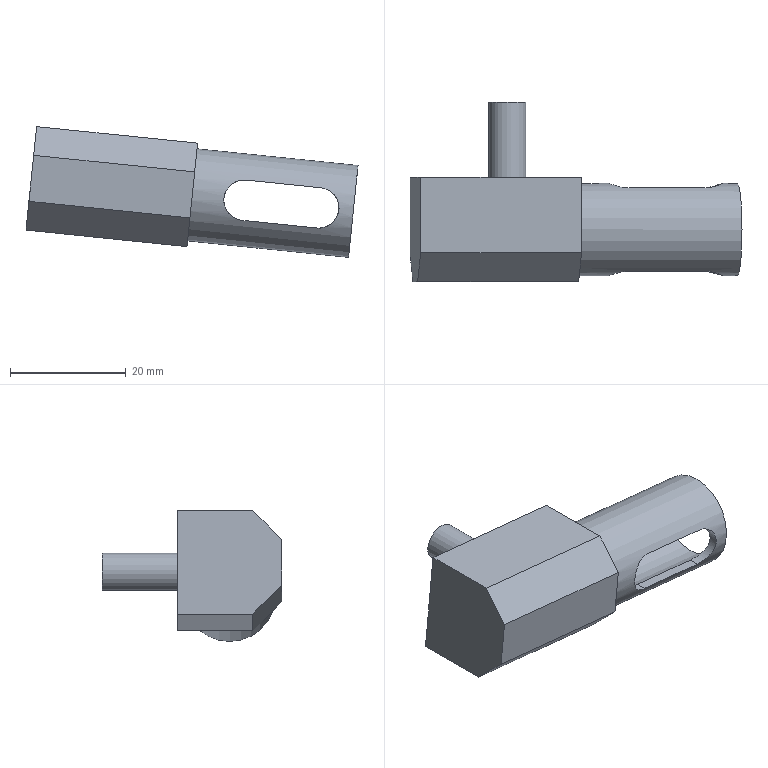Component | NX | PISTON_CYLINDER | 1 solid | 24 faces | volume 7030 mm3 | plane 16 | cylinder 8 | commonest cylinder face diameters 7 x4 16 x1 13 x1 6.5 x1 4 x1